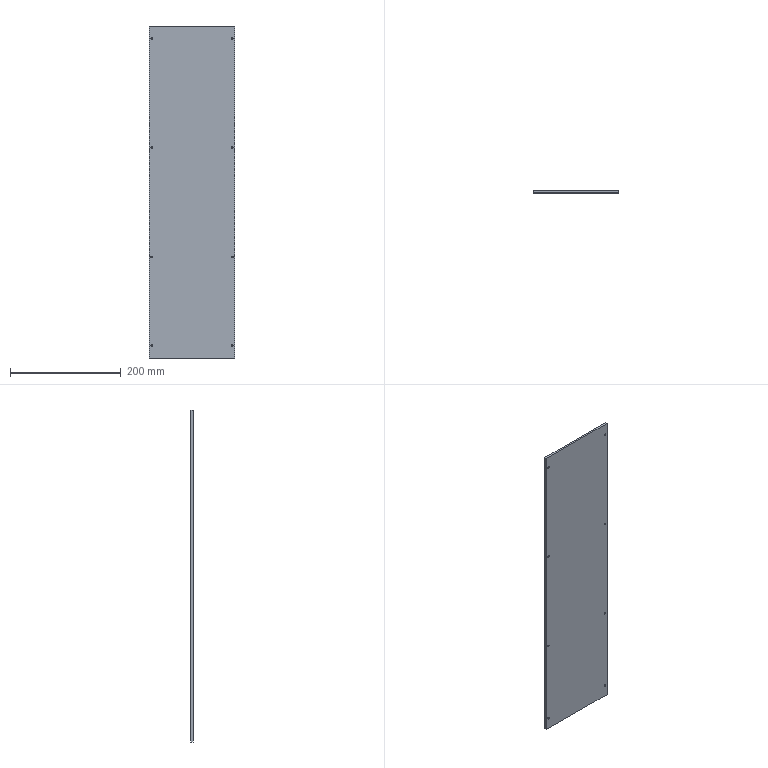Component | SolidWorks | ColumnCover-1 | 1 solid | 38 faces | box 155 x 4 x 600 mm | volume 371585 mm3 | cone 16 | cylinder 16 | plane 6 | commonest cylinder face diameters 3.4 x16
STEP:
#1=CARTESIAN_POINT('',(47.712,61.489,84.389));
#2=VERTEX_POINT('',#1);
#3=CARTESIAN_POINT('',(47.578,61.489,84.389));
#4=VERTEX_POINT('',#3);
#5=CARTESIAN_POINT('',(47.645,61.489,84.389));
#6=DIRECTION('',(-0.,1.,0.));
#7=DIRECTION('',(-1.,0.,0.));
#8=AXIS2_PLACEMENT_3D('',#5,#6,#7);
#9=CIRCLE('',#8,0.06693);
#10=EDGE_CURVE('',#2,#4,#9,.T.);
#11=ORIENTED_EDGE('',*,*,#10,.F.);
#12=CARTESIAN_POINT('',(47.771,61.548,84.389));
#13=VERTEX_POINT('',#12);
#14=CARTESIAN_POINT('',(47.771,61.548,84.389));
#15=DIRECTION('',(0.7071,0.7071,0.));
#16=VECTOR('',#15,39.37);
#17=LINE('',#14,#16);
#18=EDGE_CURVE('',#2,#13,#17,.T.);
#19=ORIENTED_EDGE('',*,*,#18,.T.);
#20=CARTESIAN_POINT('',(47.519,61.548,84.389));
#21=VERTEX_POINT('',#20);
#22=CARTESIAN_POINT('',(47.645,61.548,84.389));
#23=DIRECTION('',(-0.,1.,0.));
#24=DIRECTION('',(-1.,0.,0.));
#25=AXIS2_PLACEMENT_3D('',#22,#23,#24);
#26=CIRCLE('',#25,0.126);
#27=EDGE_CURVE('',#13,#21,#26,.T.);
#28=ORIENTED_EDGE('',*,*,#27,.T.);
#29=CARTESIAN_POINT('',(47.519,61.548,84.389));
#30=DIRECTION('',(-0.7071,0.7071,0.));
#31=VECTOR('',#30,39.37);
#32=LINE('',#29,#31);
#33=EDGE_CURVE('',#4,#21,#32,.T.);
#34=ORIENTED_EDGE('',*,*,#33,.F.);
#35=EDGE_LOOP('',(#11,#19,#28,#34));
#36=FACE_OUTER_BOUND('',#35,.T.);
#37=CARTESIAN_POINT('',(47.645,61.548,84.389));
#38=DIRECTION('',(-0.,1.,0.));
#39=DIRECTION('',(-1.,0.,0.));
#40=AXIS2_PLACEMENT_3D('',#37,#38,#39);
#41=CONICAL_SURFACE('',#40,0.126,0.7854);
#42=ADVANCED_FACE('',(#36),#41,.F.);
#43=CARTESIAN_POINT('',(47.578,61.39,84.389));
#44=VERTEX_POINT('',#43);
#45=CARTESIAN_POINT('',(47.712,61.39,84.389));
#46=VERTEX_POINT('',#45);
#47=CARTESIAN_POINT('',(47.645,61.39,84.389));
#48=DIRECTION('',(0.,-1.,-0.));
#49=DIRECTION('',(1.,0.,0.));
#50=AXIS2_PLACEMENT_3D('',#47,#48,#49);
#51=CIRCLE('',#50,0.06693);
#52=EDGE_CURVE('',#44,#46,#51,.T.);
#53=ORIENTED_EDGE('',*,*,#52,.T.);
#54=CARTESIAN_POINT('',(47.712,61.548,84.389));
#55=DIRECTION('',(-0.,1.,0.));
#56=VECTOR('',#55,39.37);
#57=LINE('',#54,#56);
#58=EDGE_CURVE('',#46,#2,#57,.T.);
#59=ORIENTED_EDGE('',*,*,#58,.T.);
#60=ORIENTED_EDGE('',*,*,#10,.T.);
#61=CARTESIAN_POINT('',(47.578,61.548,84.389));
#62=DIRECTION('',(-0.,1.,0.));
#63=VECTOR('',#62,39.37);
#64=LINE('',#61,#63);
#65=EDGE_CURVE('',#44,#4,#64,.T.);
#66=ORIENTED_EDGE('',*,*,#65,.F.);
#67=EDGE_LOOP('',(#53,#59,#60,#66));
#68=FACE_OUTER_BOUND('',#67,.T.);
#69=CARTESIAN_POINT('',(47.645,61.548,84.389));
#70=DIRECTION('',(-0.,1.,0.));
#71=DIRECTION('',(-1.,0.,0.));
#72=AXIS2_PLACEMENT_3D('',#69,#70,#71);
#73=CYLINDRICAL_SURFACE('',#72,0.06693);
#74=ADVANCED_FACE('',(#68),#73,.F.);
#75=CARTESIAN_POINT('',(42.003,61.489,84.389));
#76=VERTEX_POINT('',#75);
#77=CARTESIAN_POINT('',(41.87,61.489,84.389));
#78=VERTEX_POINT('',#77);
#79=CARTESIAN_POINT('',(41.936,61.489,84.389));
#80=DIRECTION('',(-0.,1.,0.));
#81=DIRECTION('',(-1.,0.,0.));
#82=AXIS2_PLACEMENT_3D('',#79,#80,#81);
#83=CIRCLE('',#82,0.06693);
#84=EDGE_CURVE('',#76,#78,#83,.T.);
#85=ORIENTED_EDGE('',*,*,#84,.F.);
#86=CARTESIAN_POINT('',(42.062,61.548,84.389));
#87=VERTEX_POINT('',#86);
#88=CARTESIAN_POINT('',(42.062,61.548,84.389));
#89=DIRECTION('',(0.7071,0.7071,0.));
#90=VECTOR('',#89,39.37);
#91=LINE('',#88,#90);
#92=EDGE_CURVE('',#76,#87,#91,.T.);
#93=ORIENTED_EDGE('',*,*,#92,.T.);
#94=CARTESIAN_POINT('',(41.81,61.548,84.389));
#95=VERTEX_POINT('',#94);
#96=CARTESIAN_POINT('',(41.936,61.548,84.389));
#97=DIRECTION('',(-0.,1.,0.));
#98=DIRECTION('',(-1.,0.,0.));
#99=AXIS2_PLACEMENT_3D('',#96,#97,#98);
#100=CIRCLE('',#99,0.126);
#101=EDGE_CURVE('',#87,#95,#100,.T.);
#102=ORIENTED_EDGE('',*,*,#101,.T.);
#103=CARTESIAN_POINT('',(41.81,61.548,84.389));
#104=DIRECTION('',(-0.7071,0.7071,0.));
#105=VECTOR('',#104,39.37);
#106=LINE('',#103,#105);
#107=EDGE_CURVE('',#78,#95,#106,.T.);
#108=ORIENTED_EDGE('',*,*,#107,.F.);
#109=EDGE_LOOP('',(#85,#93,#102,#108));
#110=FACE_OUTER_BOUND('',#109,.T.);
#111=CARTESIAN_POINT('',(41.936,61.548,84.389));
#112=DIRECTION('',(-0.,1.,0.));
#113=DIRECTION('',(-1.,0.,0.));
#114=AXIS2_PLACEMENT_3D('',#111,#112,#113);
#115=CONICAL_SURFACE('',#114,0.126,0.7854);
#116=ADVANCED_FACE('',(#110),#115,.F.);
#117=CARTESIAN_POINT('',(41.87,61.39,84.389));
#118=VERTEX_POINT('',#117);
#119=CARTESIAN_POINT('',(42.003,61.39,84.389));
#120=VERTEX_POINT('',#119);
#121=CARTESIAN_POINT('',(41.936,61.39,84.389));
#122=DIRECTION('',(0.,-1.,-0.));
#123=DIRECTION('',(1.,0.,0.));
#124=AXIS2_PLACEMENT_3D('',#121,#122,#123);
#125=CIRCLE('',#124,0.06693);
#126=EDGE_CURVE('',#118,#120,#125,.T.);
#127=ORIENTED_EDGE('',*,*,#126,.T.);
#128=CARTESIAN_POINT('',(42.003,61.548,84.389));
#129=DIRECTION('',(-0.,1.,0.));
#130=VECTOR('',#129,39.37);
#131=LINE('',#128,#130);
#132=EDGE_CURVE('',#120,#76,#131,.T.);
#133=ORIENTED_EDGE('',*,*,#132,.T.);
#134=ORIENTED_EDGE('',*,*,#84,.T.);
#135=CARTESIAN_POINT('',(41.87,61.548,84.389));
#136=DIRECTION('',(-0.,1.,0.));
#137=VECTOR('',#136,39.37);
#138=LINE('',#135,#137);
#139=EDGE_CURVE('',#118,#78,#138,.T.);
#140=ORIENTED_EDGE('',*,*,#139,.F.);
#141=EDGE_LOOP('',(#127,#133,#134,#140));
#142=FACE_OUTER_BOUND('',#141,.T.);
#143=CARTESIAN_POINT('',(41.936,61.548,84.389));
#144=DIRECTION('',(-0.,1.,0.));
#145=DIRECTION('',(-1.,0.,0.));
#146=AXIS2_PLACEMENT_3D('',#143,#144,#145);
#147=CYLINDRICAL_SURFACE('',#146,0.06693);
#148=ADVANCED_FACE('',(#142),#147,.F.);
#149=CARTESIAN_POINT('',(47.712,61.489,76.614));
#150=VERTEX_POINT('',#149);
#151=CARTESIAN_POINT('',(47.578,61.489,76.614));
#152=VERTEX_POINT('',#151);
#153=CARTESIAN_POINT('',(47.645,61.489,76.614));
#154=DIRECTION('',(-0.,1.,0.));
#155=DIRECTION('',(-1.,0.,0.));
#156=AXIS2_PLACEMENT_3D('',#153,#154,#155);
#157=CIRCLE('',#156,0.06693);
#158=EDGE_CURVE('',#150,#152,#157,.T.);
#159=ORIENTED_EDGE('',*,*,#158,.F.);
#160=CARTESIAN_POINT('',(47.771,61.548,76.614));
#161=VERTEX_POINT('',#160);
#162=CARTESIAN_POINT('',(47.771,61.548,76.614));
#163=DIRECTION('',(0.7071,0.7071,0.));
#164=VECTOR('',#163,39.37);
#165=LINE('',#162,#164);
#166=EDGE_CURVE('',#150,#161,#165,.T.);
#167=ORIENTED_EDGE('',*,*,#166,.T.);
#168=CARTESIAN_POINT('',(47.519,61.548,76.614));
#169=VERTEX_POINT('',#168);
#170=CARTESIAN_POINT('',(47.645,61.548,76.614));
#171=DIRECTION('',(-0.,1.,0.));
#172=DIRECTION('',(-1.,0.,0.));
#173=AXIS2_PLACEMENT_3D('',#170,#171,#172);
#174=CIRCLE('',#173,0.126);
#175=EDGE_CURVE('',#161,#169,#174,.T.);
#176=ORIENTED_EDGE('',*,*,#175,.T.);
#177=CARTESIAN_POINT('',(47.519,61.548,76.614));
#178=DIRECTION('',(-0.7071,0.7071,0.));
#179=VECTOR('',#178,39.37);
#180=LINE('',#177,#179);
#181=EDGE_CURVE('',#152,#169,#180,.T.);
#182=ORIENTED_EDGE('',*,*,#181,.F.);
#183=EDGE_LOOP('',(#159,#167,#176,#182));
#184=FACE_OUTER_BOUND('',#183,.T.);
#185=CARTESIAN_POINT('',(47.645,61.548,76.614));
#186=DIRECTION('',(-0.,1.,0.));
#187=DIRECTION('',(-1.,0.,0.));
#188=AXIS2_PLACEMENT_3D('',#185,#186,#187);
#189=CONICAL_SURFACE('',#188,0.126,0.7854);
#190=ADVANCED_FACE('',(#184),#189,.F.);
#191=CARTESIAN_POINT('',(47.578,61.39,76.614));
#192=VERTEX_POINT('',#191);
#193=CARTESIAN_POINT('',(47.712,61.39,76.614));
#194=VERTEX_POINT('',#193);
#195=CARTESIAN_POINT('',(47.645,61.39,76.614));
#196=DIRECTION('',(0.,-1.,-0.));
#197=DIRECTION('',(1.,0.,0.));
#198=AXIS2_PLACEMENT_3D('',#195,#196,#197);
#199=CIRCLE('',#198,0.06693);
#200=EDGE_CURVE('',#192,#194,#199,.T.);
#201=ORIENTED_EDGE('',*,*,#200,.T.);
#202=CARTESIAN_POINT('',(47.712,61.548,76.614));
#203=DIRECTION('',(-0.,1.,0.));
#204=VECTOR('',#203,39.37);
#205=LINE('',#202,#204);
#206=EDGE_CURVE('',#194,#150,#205,.T.);
#207=ORIENTED_EDGE('',*,*,#206,.T.);
#208=ORIENTED_EDGE('',*,*,#158,.T.);
#209=CARTESIAN_POINT('',(47.578,61.548,76.614));
#210=DIRECTION('',(-0.,1.,0.));
#211=VECTOR('',#210,39.37);
#212=LINE('',#209,#211);
#213=EDGE_CURVE('',#192,#152,#212,.T.);
#214=ORIENTED_EDGE('',*,*,#213,.F.);
#215=EDGE_LOOP('',(#201,#207,#208,#214));
#216=FACE_OUTER_BOUND('',#215,.T.);
#217=CARTESIAN_POINT('',(47.645,61.548,76.614));
#218=DIRECTION('',(-0.,1.,0.));
#219=DIRECTION('',(-1.,0.,0.));
#220=AXIS2_PLACEMENT_3D('',#217,#218,#219);
#221=CYLINDRICAL_SURFACE('',#220,0.06693);
#222=ADVANCED_FACE('',(#216),#221,.F.);
#223=CARTESIAN_POINT('',(42.003,61.489,76.614));
#224=VERTEX_POINT('',#223);
#225=CARTESIAN_POINT('',(41.87,61.489,76.614));
#226=VERTEX_POINT('',#225);
#227=CARTESIAN_POINT('',(41.936,61.489,76.614));
#228=DIRECTION('',(-0.,1.,0.));
#229=DIRECTION('',(-1.,0.,0.));
#230=AXIS2_PLACEMENT_3D('',#227,#228,#229);
#231=CIRCLE('',#230,0.06693);
#232=EDGE_CURVE('',#224,#226,#231,.T.);
#233=ORIENTED_EDGE('',*,*,#232,.F.);
#234=CARTESIAN_POINT('',(42.062,61.548,76.614));
#235=VERTEX_POINT('',#234);
#236=CARTESIAN_POINT('',(42.062,61.548,76.614));
#237=DIRECTION('',(0.7071,0.7071,0.));
#238=VECTOR('',#237,39.37);
#239=LINE('',#236,#238);
#240=EDGE_CURVE('',#224,#235,#239,.T.);
#241=ORIENTED_EDGE('',*,*,#240,.T.);
#242=CARTESIAN_POINT('',(41.81,61.548,76.614));
#243=VERTEX_POINT('',#242);
#244=CARTESIAN_POINT('',(41.936,61.548,76.614));
#245=DIRECTION('',(-0.,1.,0.));
#246=DIRECTION('',(-1.,0.,0.));
#247=AXIS2_PLACEMENT_3D('',#244,#245,#246);
#248=CIRCLE('',#247,0.126);
#249=EDGE_CURVE('',#235,#243,#248,.T.);
#250=ORIENTED_EDGE('',*,*,#249,.T.);
#251=CARTESIAN_POINT('',(41.81,61.548,76.614));
#252=DIRECTION('',(-0.7071,0.7071,0.));
#253=VECTOR('',#252,39.37);
#254=LINE('',#251,#253);
#255=EDGE_CURVE('',#226,#243,#254,.T.);
#256=ORIENTED_EDGE('',*,*,#255,.F.);
#257=EDGE_LOOP('',(#233,#241,#250,#256));
#258=FACE_OUTER_BOUND('',#257,.T.);
#259=CARTESIAN_POINT('',(41.936,61.548,76.614));
#260=DIRECTION('',(-0.,1.,0.));
#261=DIRECTION('',(-1.,0.,0.));
#262=AXIS2_PLACEMENT_3D('',#259,#260,#261);
#263=CONICAL_SURFACE('',#262,0.126,0.7854);
#264=ADVANCED_FACE('',(#258),#263,.F.);
#265=CARTESIAN_POINT('',(41.87,61.39,76.614));
#266=VERTEX_POINT('',#265);
#267=CARTESIAN_POINT('',(42.003,61.39,76.614));
#268=VERTEX_POINT('',#267);
#269=CARTESIAN_POINT('',(41.936,61.39,76.614));
#270=DIRECTION('',(0.,-1.,-0.));
#271=DIRECTION('',(1.,0.,0.));
#272=AXIS2_PLACEMENT_3D('',#269,#270,#271);
#273=CIRCLE('',#272,0.06693);
#274=EDGE_CURVE('',#266,#268,#273,.T.);
#275=ORIENTED_EDGE('',*,*,#274,.T.);
#276=CARTESIAN_POINT('',(42.003,61.548,76.614));
#277=DIRECTION('',(-0.,1.,0.));
#278=VECTOR('',#277,39.37);
#279=LINE('',#276,#278);
#280=EDGE_CURVE('',#268,#224,#279,.T.);
#281=ORIENTED_EDGE('',*,*,#280,.T.);
#282=ORIENTED_EDGE('',*,*,#232,.T.);
#283=CARTESIAN_POINT('',(41.87,61.548,76.614));
#284=DIRECTION('',(-0.,1.,0.));
#285=VECTOR('',#284,39.37);
#286=LINE('',#283,#285);
#287=EDGE_CURVE('',#266,#226,#286,.T.);
#288=ORIENTED_EDGE('',*,*,#287,.F.);
#289=EDGE_LOOP('',(#275,#281,#282,#288));
#290=FACE_OUTER_BOUND('',#289,.T.);
#291=CARTESIAN_POINT('',(41.936,61.548,76.614));
#292=DIRECTION('',(-0.,1.,0.));
#293=DIRECTION('',(-1.,0.,0.));
#294=AXIS2_PLACEMENT_3D('',#291,#292,#293);
#295=CYLINDRICAL_SURFACE('',#294,0.06693);
#296=ADVANCED_FACE('',(#290),#295,.F.);
#297=CARTESIAN_POINT('',(47.712,61.489,68.838));
#298=VERTEX_POINT('',#297);
#299=CARTESIAN_POINT('',(47.578,61.489,68.838));
#300=VERTEX_POINT('',#299);
#301=CARTESIAN_POINT('',(47.645,61.489,68.838));
#302=DIRECTION('',(-0.,1.,0.));
#303=DIRECTION('',(-1.,0.,0.));
#304=AXIS2_PLACEMENT_3D('',#301,#302,#303);
#305=CIRCLE('',#304,0.06693);
#306=EDGE_CURVE('',#298,#300,#305,.T.);
#307=ORIENTED_EDGE('',*,*,#306,.F.);
#308=CARTESIAN_POINT('',(47.771,61.548,68.838));
#309=VERTEX_POINT('',#308);
#310=CARTESIAN_POINT('',(47.771,61.548,68.838));
#311=DIRECTION('',(0.7071,0.7071,0.));
#312=VECTOR('',#311,39.37);
#313=LINE('',#310,#312);
#314=EDGE_CURVE('',#298,#309,#313,.T.);
#315=ORIENTED_EDGE('',*,*,#314,.T.);
#316=CARTESIAN_POINT('',(47.519,61.548,68.838));
#317=VERTEX_POINT('',#316);
#318=CARTESIAN_POINT('',(47.645,61.548,68.838));
#319=DIRECTION('',(-0.,1.,0.));
#320=DIRECTION('',(-1.,0.,0.));
#321=AXIS2_PLACEMENT_3D('',#318,#319,#320);
#322=CIRCLE('',#321,0.126);
#323=EDGE_CURVE('',#309,#317,#322,.T.);
#324=ORIENTED_EDGE('',*,*,#323,.T.);
#325=CARTESIAN_POINT('',(47.519,61.548,68.838));
#326=DIRECTION('',(-0.7071,0.7071,0.));
#327=VECTOR('',#326,39.37);
#328=LINE('',#325,#327);
#329=EDGE_CURVE('',#300,#317,#328,.T.);
#330=ORIENTED_EDGE('',*,*,#329,.F.);
#331=EDGE_LOOP('',(#307,#315,#324,#330));
#332=FACE_OUTER_BOUND('',#331,.T.);
#333=CARTESIAN_POINT('',(47.645,61.548,68.838));
#334=DIRECTION('',(-0.,1.,0.));
#335=DIRECTION('',(-1.,0.,0.));
#336=AXIS2_PLACEMENT_3D('',#333,#334,#335);
#337=CONICAL_SURFACE('',#336,0.126,0.7854);
#338=ADVANCED_FACE('',(#332),#337,.F.);
#339=CARTESIAN_POINT('',(47.578,61.39,68.838));
#340=VERTEX_POINT('',#339);
#341=CARTESIAN_POINT('',(47.712,61.39,68.838));
#342=VERTEX_POINT('',#341);
#343=CARTESIAN_POINT('',(47.645,61.39,68.838));
#344=DIRECTION('',(0.,-1.,-0.));
#345=DIRECTION('',(1.,0.,0.));
#346=AXIS2_PLACEMENT_3D('',#343,#344,#345);
#347=CIRCLE('',#346,0.06693);
#348=EDGE_CURVE('',#340,#342,#347,.T.);
#349=ORIENTED_EDGE('',*,*,#348,.T.);
#350=CARTESIAN_POINT('',(47.712,61.548,68.838));
#351=DIRECTION('',(-0.,1.,0.));
#352=VECTOR('',#351,39.37);
#353=LINE('',#350,#352);
#354=EDGE_CURVE('',#342,#298,#353,.T.);
#355=ORIENTED_EDGE('',*,*,#354,.T.);
#356=ORIENTED_EDGE('',*,*,#306,.T.);
#357=CARTESIAN_POINT('',(47.578,61.548,68.838));
#358=DIRECTION('',(-0.,1.,0.));
#359=VECTOR('',#358,39.37);
#360=LINE('',#357,#359);
#361=EDGE_CURVE('',#340,#300,#360,.T.);
#362=ORIENTED_EDGE('',*,*,#361,.F.);
#363=EDGE_LOOP('',(#349,#355,#356,#362));
#364=FACE_OUTER_BOUND('',#363,.T.);
#365=CARTESIAN_POINT('',(47.645,61.548,68.838));
#366=DIRECTION('',(-0.,1.,0.));
#367=DIRECTION('',(-1.,0.,0.));
#368=AXIS2_PLACEMENT_3D('',#365,#366,#367);
#369=CYLINDRICAL_SURFACE('',#368,0.06693);
#370=ADVANCED_FACE('',(#364),#369,.F.);
#371=CARTESIAN_POINT('',(42.003,61.489,68.838));
#372=VERTEX_POINT('',#371);
#373=CARTESIAN_POINT('',(41.87,61.489,68.838));
#374=VERTEX_POINT('',#373);
#375=CARTESIAN_POINT('',(41.936,61.489,68.838));
#376=DIRECTION('',(-0.,1.,0.));
#377=DIRECTION('',(-1.,0.,0.));
#378=AXIS2_PLACEMENT_3D('',#375,#376,#377);
#379=CIRCLE('',#378,0.06693);
#380=EDGE_CURVE('',#372,#374,#379,.T.);
#381=ORIENTED_EDGE('',*,*,#380,.F.);
#382=CARTESIAN_POINT('',(42.062,61.548,68.838));
#383=VERTEX_POINT('',#382);
#384=CARTESIAN_POINT('',(42.062,61.548,68.838));
#385=DIRECTION('',(0.7071,0.7071,0.));
#386=VECTOR('',#385,39.37);
#387=LINE('',#384,#386);
#388=EDGE_CURVE('',#372,#383,#387,.T.);
#389=ORIENTED_EDGE('',*,*,#388,.T.);
#390=CARTESIAN_POINT('',(41.81,61.548,68.838));
#391=VERTEX_POINT('',#390);
#392=CARTESIAN_POINT('',(41.936,61.548,68.838));
#393=DIRECTION('',(-0.,1.,0.));
#394=DIRECTION('',(-1.,0.,0.));
#395=AXIS2_PLACEMENT_3D('',#392,#393,#394);
#396=CIRCLE('',#395,0.126);
#397=EDGE_CURVE('',#383,#391,#396,.T.);
#398=ORIENTED_EDGE('',*,*,#397,.T.);
#399=CARTESIAN_POINT('',(41.81,61.548,68.838));
#400=DIRECTION('',(-0.7071,0.7071,0.));
#401=VECTOR('',#400,39.37);
#402=LINE('',#399,#401);
#403=EDGE_CURVE('',#374,#391,#402,.T.);
#404=ORIENTED_EDGE('',*,*,#403,.F.);
#405=EDGE_LOOP('',(#381,#389,#398,#404));
#406=FACE_OUTER_BOUND('',#405,.T.);
#407=CARTESIAN_POINT('',(41.936,61.548,68.838));
#408=DIRECTION('',(-0.,1.,0.));
#409=DIRECTION('',(-1.,0.,0.));
#410=AXIS2_PLACEMENT_3D('',#407,#408,#409);
#411=CONICAL_SURFACE('',#410,0.126,0.7854);
#412=ADVANCED_FACE('',(#406),#411,.F.);
#413=CARTESIAN_POINT('',(41.87,61.39,68.838));
#414=VERTEX_POINT('',#413);
#415=CARTESIAN_POINT('',(42.003,61.39,68.838));
#416=VERTEX_POINT('',#415);
#417=CARTESIAN_POINT('',(41.936,61.39,68.838));
#418=DIRECTION('',(0.,-1.,-0.));
#419=DIRECTION('',(1.,0.,0.));
#420=AXIS2_PLACEMENT_3D('',#417,#418,#419);
#421=CIRCLE('',#420,0.06693);
#422=EDGE_CURVE('',#414,#416,#421,.T.);
#423=ORIENTED_EDGE('',*,*,#422,.T.);
#424=CARTESIAN_POINT('',(42.003,61.548,68.838));
#425=DIRECTION('',(-0.,1.,0.));
#426=VECTOR('',#425,39.37);
#427=LINE('',#424,#426);
#428=EDGE_CURVE('',#416,#372,#427,.T.);
#429=ORIENTED_EDGE('',*,*,#428,.T.);
#430=ORIENTED_EDGE('',*,*,#380,.T.);
#431=CARTESIAN_POINT('',(41.87,61.548,68.838));
#432=DIRECTION('',(-0.,1.,0.));
#433=VECTOR('',#432,39.37);
#434=LINE('',#431,#433);
#435=EDGE_CURVE('',#414,#374,#434,.T.);
#436=ORIENTED_EDGE('',*,*,#435,.F.);
#437=EDGE_LOOP('',(#423,#429,#430,#436));
#438=FACE_OUTER_BOUND('',#437,.T.);
#439=CARTESIAN_POINT('',(41.936,61.548,68.838));
#440=DIRECTION('',(-0.,1.,0.));
#441=DIRECTION('',(-1.,0.,0.));
#442=AXIS2_PLACEMENT_3D('',#439,#440,#441);
#443=CYLINDRICAL_SURFACE('',#442,0.06693);
#444=ADVANCED_FACE('',(#438),#443,.F.);
#445=CARTESIAN_POINT('',(47.712,61.489,62.539));
#446=VERTEX_POINT('',#445);
#447=CARTESIAN_POINT('',(47.578,61.489,62.539));
#448=VERTEX_POINT('',#447);
#449=CARTESIAN_POINT('',(47.645,61.489,62.539));
#450=DIRECTION('',(-0.,1.,0.));
#451=DIRECTION('',(-1.,0.,0.));
#452=AXIS2_PLACEMENT_3D('',#449,#450,#451);
#453=CIRCLE('',#452,0.06693);
#454=EDGE_CURVE('',#446,#448,#453,.T.);
#455=ORIENTED_EDGE('',*,*,#454,.F.);
#456=CARTESIAN_POINT('',(47.771,61.548,62.539));
#457=VERTEX_POINT('',#456);
#458=CARTESIAN_POINT('',(47.771,61.548,62.539));
#459=DIRECTION('',(0.7071,0.7071,0.));
#460=VECTOR('',#459,39.37);
#461=LINE('',#458,#460);
#462=EDGE_CURVE('',#446,#457,#461,.T.);
#463=ORIENTED_EDGE('',*,*,#462,.T.);
#464=CARTESIAN_POINT('',(47.519,61.548,62.539));
#465=VERTEX_POINT('',#464);
#466=CARTESIAN_POINT('',(47.645,61.548,62.539));
#467=DIRECTION('',(-0.,1.,0.));
#468=DIRECTION('',(-1.,0.,0.));
#469=AXIS2_PLACEMENT_3D('',#466,#467,#468);
#470=CIRCLE('',#469,0.126);
#471=EDGE_CURVE('',#457,#465,#470,.T.);
#472=ORIENTED_EDGE('',*,*,#471,.T.);
#473=CARTESIAN_POINT('',(47.519,61.548,62.539));
#474=DIRECTION('',(-0.7071,0.7071,0.));
#475=VECTOR('',#474,39.37);
#476=LINE('',#473,#475);
#477=EDGE_CURVE('',#448,#465,#476,.T.);
#478=ORIENTED_EDGE('',*,*,#477,.F.);
#479=EDGE_LOOP('',(#455,#463,#472,#478));
#480=FACE_OUTER_BOUND('',#479,.T.);
#481=CARTESIAN_POINT('',(47.645,61.548,62.539));
#482=DIRECTION('',(-0.,1.,0.));
#483=DIRECTION('',(-1.,0.,0.));
#484=AXIS2_PLACEMENT_3D('',#481,#482,#483);
#485=CONICAL_SURFACE('',#484,0.126,0.7854);
#486=ADVANCED_FACE('',(#480),#485,.F.);
#487=CARTESIAN_POINT('',(47.578,61.39,62.539));
#488=VERTEX_POINT('',#487);
#489=CARTESIAN_POINT('',(47.712,61.39,62.539));
#490=VERTEX_POINT('',#489);
#491=CARTESIAN_POINT('',(47.645,61.39,62.539));
#492=DIRECTION('',(0.,-1.,-0.));
#493=DIRECTION('',(1.,0.,0.));
#494=AXIS2_PLACEMENT_3D('',#491,#492,#493);
#495=CIRCLE('',#494,0.06693);
#496=EDGE_CURVE('',#488,#490,#495,.T.);
#497=ORIENTED_EDGE('',*,*,#496,.T.);
#498=CARTESIAN_POINT('',(47.712,61.548,62.539));
#499=DIRECTION('',(-0.,1.,0.));
#500=VECTOR('',#499,39.37);
#501=LINE('',#498,#500);
#502=EDGE_CURVE('',#490,#446,#501,.T.);
#503=ORIENTED_EDGE('',*,*,#502,.T.);
#504=ORIENTED_EDGE('',*,*,#454,.T.);
#505=CARTESIAN_POINT('',(47.578,61.548,62.539));
#506=DIRECTION('',(-0.,1.,0.));
#507=VECTOR('',#506,39.37);
#508=LINE('',#505,#507);
#509=EDGE_CURVE('',#488,#448,#508,.T.);
#510=ORIENTED_EDGE('',*,*,#509,.F.);
#511=EDGE_LOOP('',(#497,#503,#504,#510));
#512=FACE_OUTER_BOUND('',#511,.T.);
#513=CARTESIAN_POINT('',(47.645,61.548,62.539));
#514=DIRECTION('',(-0.,1.,0.));
#515=DIRECTION('',(-1.,0.,0.));
#516=AXIS2_PLACEMENT_3D('',#513,#514,#515);
#517=CYLINDRICAL_SURFACE('',#516,0.06693);
#518=ADVANCED_FACE('',(#512),#517,.F.);
#519=CARTESIAN_POINT('',(42.003,61.489,62.539));
#520=VERTEX_POINT('',#519);
#521=CARTESIAN_POINT('',(41.87,61.489,62.539));
#522=VERTEX_POINT('',#521);
#523=CARTESIAN_POINT('',(41.936,61.489,62.539));
#524=DIRECTION('',(-0.,1.,0.));
#525=DIRECTION('',(-1.,0.,0.));
#526=AXIS2_PLACEMENT_3D('',#523,#524,#525);
#527=CIRCLE('',#526,0.06693);
#528=EDGE_CURVE('',#520,#522,#527,.T.);
#529=ORIENTED_EDGE('',*,*,#528,.F.);
#530=CARTESIAN_POINT('',(42.062,61.548,62.539));
#531=VERTEX_POINT('',#530);
#532=CARTESIAN_POINT('',(42.062,61.548,62.539));
#533=DIRECTION('',(0.7071,0.7071,0.));
#534=VECTOR('',#533,39.37);
#535=LINE('',#532,#534);
#536=EDGE_CURVE('',#520,#531,#535,.T.);
#537=ORIENTED_EDGE('',*,*,#536,.T.);
#538=CARTESIAN_POINT('',(41.81,61.548,62.539));
#539=VERTEX_POINT('',#538);
#540=CARTESIAN_POINT('',(41.936,61.548,62.539));
#541=DIRECTION('',(-0.,1.,0.));
#542=DIRECTION('',(-1.,0.,0.));
#543=AXIS2_PLACEMENT_3D('',#540,#541,#542);
#544=CIRCLE('',#543,0.126);
#545=EDGE_CURVE('',#531,#539,#544,.T.);
#546=ORIENTED_EDGE('',*,*,#545,.T.);
#547=CARTESIAN_POINT('',(41.81,61.548,62.539));
#548=DIRECTION('',(-0.7071,0.7071,0.));
#549=VECTOR('',#548,39.37);
#550=LINE('',#547,#549);
#551=EDGE_CURVE('',#522,#539,#550,.T.);
#552=ORIENTED_EDGE('',*,*,#551,.F.);
#553=EDGE_LOOP('',(#529,#537,#546,#552));
#554=FACE_OUTER_BOUND('',#553,.T.);
#555=CARTESIAN_POINT('',(41.936,61.548,62.539));
#556=DIRECTION('',(-0.,1.,0.));
#557=DIRECTION('',(-1.,0.,0.));
#558=AXIS2_PLACEMENT_3D('',#555,#556,#557);
#559=CONICAL_SURFACE('',#558,0.126,0.7854);
#560=ADVANCED_FACE('',(#554),#559,.F.);
#561=CARTESIAN_POINT('',(41.87,61.39,62.539));
#562=VERTEX_POINT('',#561);
#563=CARTESIAN_POINT('',(42.003,61.39,62.539));
#564=VERTEX_POINT('',#563);
#565=CARTESIAN_POINT('',(41.936,61.39,62.539));
#566=DIRECTION('',(0.,-1.,-0.));
#567=DIRECTION('',(1.,0.,0.));
#568=AXIS2_PLACEMENT_3D('',#565,#566,#567);
#569=CIRCLE('',#568,0.06693);
#570=EDGE_CURVE('',#562,#564,#569,.T.);
#571=ORIENTED_EDGE('',*,*,#570,.T.);
#572=CARTESIAN_POINT('',(42.003,61.548,62.539));
#573=DIRECTION('',(-0.,1.,0.));
#574=VECTOR('',#573,39.37);
#575=LINE('',#572,#574);
#576=EDGE_CURVE('',#564,#520,#575,.T.);
#577=ORIENTED_EDGE('',*,*,#576,.T.);
#578=ORIENTED_EDGE('',*,*,#528,.T.);
#579=CARTESIAN_POINT('',(41.87,61.548,62.539));
#580=DIRECTION('',(-0.,1.,0.));
#581=VECTOR('',#580,39.37);
#582=LINE('',#579,#581);
#583=EDGE_CURVE('',#562,#522,#582,.T.);
#584=ORIENTED_EDGE('',*,*,#583,.F.);
#585=EDGE_LOOP('',(#571,#577,#578,#584));
#586=FACE_OUTER_BOUND('',#585,.T.);
#587=CARTESIAN_POINT('',(41.936,61.548,62.539));
#588=DIRECTION('',(-0.,1.,0.));
#589=DIRECTION('',(-1.,0.,0.));
#590=AXIS2_PLACEMENT_3D('',#587,#588,#589);
#591=CYLINDRICAL_SURFACE('',#590,0.06693);
#592=ADVANCED_FACE('',(#586),#591,.F.);
#593=CARTESIAN_POINT('',(41.74,61.39,61.653));
#594=VERTEX_POINT('',#593);
#595=CARTESIAN_POINT('',(41.74,61.39,85.275));
#596=VERTEX_POINT('',#595);
#597=CARTESIAN_POINT('',(41.74,61.39,61.653));
#598=DIRECTION('',(0.,-0.,1.));
#599=VECTOR('',#598,39.37);
#600=LINE('',#597,#599);
#601=EDGE_CURVE('',#594,#596,#600,.T.);
#602=ORIENTED_EDGE('',*,*,#601,.T.);
#603=CARTESIAN_POINT('',(41.74,61.548,85.275));
#604=VERTEX_POINT('',#603);
#605=CARTESIAN_POINT('',(41.74,61.548,85.275));
#606=DIRECTION('',(0.,-1.,-0.));
#607=VECTOR('',#606,39.37);
#608=LINE('',#605,#607);
#609=EDGE_CURVE('',#604,#596,#608,.T.);
#610=ORIENTED_EDGE('',*,*,#609,.F.);
#611=CARTESIAN_POINT('',(41.74,61.548,61.653));
#612=VERTEX_POINT('',#611);
#613=CARTESIAN_POINT('',(41.74,61.548,61.653));
#614=DIRECTION('',(0.,-0.,1.));
#615=VECTOR('',#614,39.37);
#616=LINE('',#613,#615);
#617=EDGE_CURVE('',#612,#604,#616,.T.);
#618=ORIENTED_EDGE('',*,*,#617,.F.);
#619=CARTESIAN_POINT('',(41.74,61.548,61.653));
#620=DIRECTION('',(0.,-1.,-0.));
#621=VECTOR('',#620,39.37);
#622=LINE('',#619,#621);
#623=EDGE_CURVE('',#612,#594,#622,.T.);
#624=ORIENTED_EDGE('',*,*,#623,.T.);
#625=EDGE_LOOP('',(#602,#610,#618,#624));
#626=FACE_OUTER_BOUND('',#625,.T.);
#627=CARTESIAN_POINT('',(41.74,61.548,61.653));
#628=DIRECTION('',(1.,0.,0.));
#629=DIRECTION('',(-0.,1.,0.));
#630=AXIS2_PLACEMENT_3D('',#627,#628,#629);
#631=PLANE('',#630);
#632=ADVANCED_FACE('',(#626),#631,.F.);
#633=CARTESIAN_POINT('',(47.842,61.39,85.275));
#634=VERTEX_POINT('',#633);
#635=CARTESIAN_POINT('',(47.842,61.39,85.275));
#636=DIRECTION('',(1.,-0.,0.));
#637=VECTOR('',#636,39.37);
#638=LINE('',#635,#637);
#639=EDGE_CURVE('',#596,#634,#638,.T.);
#640=ORIENTED_EDGE('',*,*,#639,.T.);
#641=CARTESIAN_POINT('',(47.842,61.548,85.275));
#642=VERTEX_POINT('',#641);
#643=CARTESIAN_POINT('',(47.842,61.548,85.275));
#644=DIRECTION('',(0.,-1.,-0.));
#645=VECTOR('',#644,39.37);
#646=LINE('',#643,#645);
#647=EDGE_CURVE('',#642,#634,#646,.T.);
#648=ORIENTED_EDGE('',*,*,#647,.F.);
#649=CARTESIAN_POINT('',(47.842,61.548,85.275));
#650=DIRECTION('',(1.,-0.,0.));
#651=VECTOR('',#650,39.37);
#652=LINE('',#649,#651);
#653=EDGE_CURVE('',#604,#642,#652,.T.);
#654=ORIENTED_EDGE('',*,*,#653,.F.);
#655=ORIENTED_EDGE('',*,*,#609,.T.);
#656=EDGE_LOOP('',(#640,#648,#654,#655));
#657=FACE_OUTER_BOUND('',#656,.T.);
#658=CARTESIAN_POINT('',(47.842,61.548,85.275));
#659=DIRECTION('',(-0.,0.,-1.));
#660=DIRECTION('',(0.,-1.,-0.));
#661=AXIS2_PLACEMENT_3D('',#658,#659,#660);
#662=PLANE('',#661);
#663=ADVANCED_FACE('',(#657),#662,.F.);
#664=CARTESIAN_POINT('',(47.842,61.39,61.653));
#665=VERTEX_POINT('',#664);
#666=CARTESIAN_POINT('',(47.842,61.39,61.653));
#667=DIRECTION('',(-0.,0.,-1.));
#668=VECTOR('',#667,39.37);
#669=LINE('',#666,#668);
#670=EDGE_CURVE('',#634,#665,#669,.T.);
#671=ORIENTED_EDGE('',*,*,#670,.T.);
#672=CARTESIAN_POINT('',(47.842,61.548,61.653));
#673=VERTEX_POINT('',#672);
#674=CARTESIAN_POINT('',(47.842,61.548,61.653));
#675=DIRECTION('',(0.,-1.,-0.));
#676=VECTOR('',#675,39.37);
#677=LINE('',#674,#676);
#678=EDGE_CURVE('',#673,#665,#677,.T.);
#679=ORIENTED_EDGE('',*,*,#678,.F.);
#680=CARTESIAN_POINT('',(47.842,61.548,61.653));
#681=DIRECTION('',(-0.,0.,-1.));
#682=VECTOR('',#681,39.37);
#683=LINE('',#680,#682);
#684=EDGE_CURVE('',#642,#673,#683,.T.);
#685=ORIENTED_EDGE('',*,*,#684,.F.);
#686=ORIENTED_EDGE('',*,*,#647,.T.);
#687=EDGE_LOOP('',(#671,#679,#685,#686));
#688=FACE_OUTER_BOUND('',#687,.T.);
#689=CARTESIAN_POINT('',(47.842,61.548,61.653));
#690=DIRECTION('',(-1.,-0.,-0.));
#691=DIRECTION('',(0.,-1.,-0.));
#692=AXIS2_PLACEMENT_3D('',#689,#690,#691);
#693=PLANE('',#692);
#694=ADVANCED_FACE('',(#688),#693,.F.);
#695=CARTESIAN_POINT('',(47.842,61.39,61.653));
#696=DIRECTION('',(-1.,0.,-0.));
#697=VECTOR('',#696,39.37);
#698=LINE('',#695,#697);
#699=EDGE_CURVE('',#665,#594,#698,.T.);
#700=ORIENTED_EDGE('',*,*,#699,.T.);
#701=ORIENTED_EDGE('',*,*,#623,.F.);
#702=CARTESIAN_POINT('',(47.842,61.548,61.653));
#703=DIRECTION('',(-1.,0.,-0.));
#704=VECTOR('',#703,39.37);
#705=LINE('',#702,#704);
#706=EDGE_CURVE('',#673,#612,#705,.T.);
#707=ORIENTED_EDGE('',*,*,#706,.F.);
#708=ORIENTED_EDGE('',*,*,#678,.T.);
#709=EDGE_LOOP('',(#700,#701,#707,#708));
#710=FACE_OUTER_BOUND('',#709,.T.);
#711=CARTESIAN_POINT('',(47.842,61.548,61.653));
#712=DIRECTION('',(0.,-0.,1.));
#713=DIRECTION('',(-0.,1.,0.));
#714=AXIS2_PLACEMENT_3D('',#711,#712,#713);
#715=PLANE('',#714);
#716=ADVANCED_FACE('',(#710),#715,.F.);
#717=CARTESIAN_POINT('',(47.645,61.548,84.389));
#718=DIRECTION('',(-0.,1.,0.));
#719=DIRECTION('',(-1.,0.,0.));
#720=AXIS2_PLACEMENT_3D('',#717,#718,#719);
#721=CIRCLE('',#720,0.126);
#722=EDGE_CURVE('',#21,#13,#721,.T.);
#723=ORIENTED_EDGE('',*,*,#722,.F.);
#724=ORIENTED_EDGE('',*,*,#27,.F.);
#725=EDGE_LOOP('',(#723,#724));
#726=FACE_BOUND('',#725,.T.);
#727=CARTESIAN_POINT('',(41.936,61.548,84.389));
#728=DIRECTION('',(-0.,1.,0.));
#729=DIRECTION('',(-1.,0.,0.));
#730=AXIS2_PLACEMENT_3D('',#727,#728,#729);
#731=CIRCLE('',#730,0.126);
#732=EDGE_CURVE('',#95,#87,#731,.T.);
#733=ORIENTED_EDGE('',*,*,#732,.F.);
#734=ORIENTED_EDGE('',*,*,#101,.F.);
#735=EDGE_LOOP('',(#733,#734));
#736=FACE_BOUND('',#735,.T.);
#737=CARTESIAN_POINT('',(47.645,61.548,76.614));
#738=DIRECTION('',(-0.,1.,0.));
#739=DIRECTION('',(-1.,0.,0.));
#740=AXIS2_PLACEMENT_3D('',#737,#738,#739);
#741=CIRCLE('',#740,0.126);
#742=EDGE_CURVE('',#169,#161,#741,.T.);
#743=ORIENTED_EDGE('',*,*,#742,.F.);
#744=ORIENTED_EDGE('',*,*,#175,.F.);
#745=EDGE_LOOP('',(#743,#744));
#746=FACE_BOUND('',#745,.T.);
#747=CARTESIAN_POINT('',(41.936,61.548,76.614));
#748=DIRECTION('',(-0.,1.,0.));
#749=DIRECTION('',(-1.,0.,0.));
#750=AXIS2_PLACEMENT_3D('',#747,#748,#749);
#751=CIRCLE('',#750,0.126);
#752=EDGE_CURVE('',#243,#235,#751,.T.);
#753=ORIENTED_EDGE('',*,*,#752,.F.);
#754=ORIENTED_EDGE('',*,*,#249,.F.);
#755=EDGE_LOOP('',(#753,#754));
#756=FACE_BOUND('',#755,.T.);
#757=CARTESIAN_POINT('',(47.645,61.548,68.838));
#758=DIRECTION('',(-0.,1.,0.));
#759=DIRECTION('',(-1.,0.,0.));
#760=AXIS2_PLACEMENT_3D('',#757,#758,#759);
#761=CIRCLE('',#760,0.126);
#762=EDGE_CURVE('',#317,#309,#761,.T.);
#763=ORIENTED_EDGE('',*,*,#762,.F.);
#764=ORIENTED_EDGE('',*,*,#323,.F.);
#765=EDGE_LOOP('',(#763,#764));
#766=FACE_BOUND('',#765,.T.);
#767=CARTESIAN_POINT('',(41.936,61.548,68.838));
#768=DIRECTION('',(-0.,1.,0.));
#769=DIRECTION('',(-1.,0.,0.));
#770=AXIS2_PLACEMENT_3D('',#767,#768,#769);
#771=CIRCLE('',#770,0.126);
#772=EDGE_CURVE('',#391,#383,#771,.T.);
#773=ORIENTED_EDGE('',*,*,#772,.F.);
#774=ORIENTED_EDGE('',*,*,#397,.F.);
#775=EDGE_LOOP('',(#773,#774));
#776=FACE_BOUND('',#775,.T.);
#777=CARTESIAN_POINT('',(47.645,61.548,62.539));
#778=DIRECTION('',(-0.,1.,0.));
#779=DIRECTION('',(-1.,0.,0.));
#780=AXIS2_PLACEMENT_3D('',#777,#778,#779);
#781=CIRCLE('',#780,0.126);
#782=EDGE_CURVE('',#465,#457,#781,.T.);
#783=ORIENTED_EDGE('',*,*,#782,.F.);
#784=ORIENTED_EDGE('',*,*,#471,.F.);
#785=EDGE_LOOP('',(#783,#784));
#786=FACE_BOUND('',#785,.T.);
#787=CARTESIAN_POINT('',(41.936,61.548,62.539));
#788=DIRECTION('',(-0.,1.,0.));
#789=DIRECTION('',(-1.,0.,0.));
#790=AXIS2_PLACEMENT_3D('',#787,#788,#789);
#791=CIRCLE('',#790,0.126);
#792=EDGE_CURVE('',#539,#531,#791,.T.);
#793=ORIENTED_EDGE('',*,*,#792,.F.);
#794=ORIENTED_EDGE('',*,*,#545,.F.);
#795=EDGE_LOOP('',(#793,#794));
#796=FACE_BOUND('',#795,.T.);
#797=ORIENTED_EDGE('',*,*,#617,.T.);
#798=ORIENTED_EDGE('',*,*,#653,.T.);
#799=ORIENTED_EDGE('',*,*,#684,.T.);
#800=ORIENTED_EDGE('',*,*,#706,.T.);
#801=EDGE_LOOP('',(#797,#798,#799,#800));
#802=FACE_OUTER_BOUND('',#801,.T.);
#803=CARTESIAN_POINT('',(44.791,61.548,73.464));
#804=DIRECTION('',(-0.,-1.,-0.));
#805=DIRECTION('',(1.,-0.,0.));
#806=AXIS2_PLACEMENT_3D('',#803,#804,#805);
#807=PLANE('',#806);
#808=ADVANCED_FACE('',(#726,#736,#746,#756,#766,#776,#786,#796,#802),#807,.F.);
#809=ORIENTED_EDGE('',*,*,#52,.F.);
#810=CARTESIAN_POINT('',(47.645,61.39,84.389));
#811=DIRECTION('',(0.,-1.,-0.));
#812=DIRECTION('',(1.,0.,0.));
#813=AXIS2_PLACEMENT_3D('',#810,#811,#812);
#814=CIRCLE('',#813,0.06693);
#815=EDGE_CURVE('',#46,#44,#814,.T.);
#816=ORIENTED_EDGE('',*,*,#815,.F.);
#817=EDGE_LOOP('',(#809,#816));
#818=FACE_BOUND('',#817,.T.);
#819=ORIENTED_EDGE('',*,*,#126,.F.);
#820=CARTESIAN_POINT('',(41.936,61.39,84.389));
#821=DIRECTION('',(0.,-1.,-0.));
#822=DIRECTION('',(1.,0.,0.));
#823=AXIS2_PLACEMENT_3D('',#820,#821,#822);
#824=CIRCLE('',#823,0.06693);
#825=EDGE_CURVE('',#120,#118,#824,.T.);
#826=ORIENTED_EDGE('',*,*,#825,.F.);
#827=EDGE_LOOP('',(#819,#826));
#828=FACE_BOUND('',#827,.T.);
#829=ORIENTED_EDGE('',*,*,#200,.F.);
#830=CARTESIAN_POINT('',(47.645,61.39,76.614));
#831=DIRECTION('',(0.,-1.,-0.));
#832=DIRECTION('',(1.,0.,0.));
#833=AXIS2_PLACEMENT_3D('',#830,#831,#832);
#834=CIRCLE('',#833,0.06693);
#835=EDGE_CURVE('',#194,#192,#834,.T.);
#836=ORIENTED_EDGE('',*,*,#835,.F.);
#837=EDGE_LOOP('',(#829,#836));
#838=FACE_BOUND('',#837,.T.);
#839=ORIENTED_EDGE('',*,*,#274,.F.);
#840=CARTESIAN_POINT('',(41.936,61.39,76.614));
#841=DIRECTION('',(0.,-1.,-0.));
#842=DIRECTION('',(1.,0.,0.));
#843=AXIS2_PLACEMENT_3D('',#840,#841,#842);
#844=CIRCLE('',#843,0.06693);
#845=EDGE_CURVE('',#268,#266,#844,.T.);
#846=ORIENTED_EDGE('',*,*,#845,.F.);
#847=EDGE_LOOP('',(#839,#846));
#848=FACE_BOUND('',#847,.T.);
#849=ORIENTED_EDGE('',*,*,#348,.F.);
#850=CARTESIAN_POINT('',(47.645,61.39,68.838));
#851=DIRECTION('',(0.,-1.,-0.));
#852=DIRECTION('',(1.,0.,0.));
#853=AXIS2_PLACEMENT_3D('',#850,#851,#852);
#854=CIRCLE('',#853,0.06693);
#855=EDGE_CURVE('',#342,#340,#854,.T.);
#856=ORIENTED_EDGE('',*,*,#855,.F.);
#857=EDGE_LOOP('',(#849,#856));
#858=FACE_BOUND('',#857,.T.);
#859=ORIENTED_EDGE('',*,*,#422,.F.);
#860=CARTESIAN_POINT('',(41.936,61.39,68.838));
#861=DIRECTION('',(0.,-1.,-0.));
#862=DIRECTION('',(1.,0.,0.));
#863=AXIS2_PLACEMENT_3D('',#860,#861,#862);
#864=CIRCLE('',#863,0.06693);
#865=EDGE_CURVE('',#416,#414,#864,.T.);
#866=ORIENTED_EDGE('',*,*,#865,.F.);
#867=EDGE_LOOP('',(#859,#866));
#868=FACE_BOUND('',#867,.T.);
#869=ORIENTED_EDGE('',*,*,#496,.F.);
#870=CARTESIAN_POINT('',(47.645,61.39,62.539));
#871=DIRECTION('',(0.,-1.,-0.));
#872=DIRECTION('',(1.,0.,0.));
#873=AXIS2_PLACEMENT_3D('',#870,#871,#872);
#874=CIRCLE('',#873,0.06693);
#875=EDGE_CURVE('',#490,#488,#874,.T.);
#876=ORIENTED_EDGE('',*,*,#875,.F.);
#877=EDGE_LOOP('',(#869,#876));
#878=FACE_BOUND('',#877,.T.);
#879=ORIENTED_EDGE('',*,*,#570,.F.);
#880=CARTESIAN_POINT('',(41.936,61.39,62.539));
#881=DIRECTION('',(0.,-1.,-0.));
#882=DIRECTION('',(1.,0.,0.));
#883=AXIS2_PLACEMENT_3D('',#880,#881,#882);
#884=CIRCLE('',#883,0.06693);
#885=EDGE_CURVE('',#564,#562,#884,.T.);
#886=ORIENTED_EDGE('',*,*,#885,.F.);
#887=EDGE_LOOP('',(#879,#886));
#888=FACE_BOUND('',#887,.T.);
#889=ORIENTED_EDGE('',*,*,#601,.F.);
#890=ORIENTED_EDGE('',*,*,#699,.F.);
#891=ORIENTED_EDGE('',*,*,#670,.F.);
#892=ORIENTED_EDGE('',*,*,#639,.F.);
#893=EDGE_LOOP('',(#889,#890,#891,#892));
#894=FACE_OUTER_BOUND('',#893,.T.);
#895=CARTESIAN_POINT('',(44.791,61.39,73.464));
#896=DIRECTION('',(-0.,-1.,-0.));
#897=DIRECTION('',(1.,-0.,0.));
#898=AXIS2_PLACEMENT_3D('',#895,#896,#897);
#899=PLANE('',#898);
#900=ADVANCED_FACE('',(#818,#828,#838,#848,#858,#868,#878,#888,#894),#899,.T.);
#901=ORIENTED_EDGE('',*,*,#576,.F.);
#902=ORIENTED_EDGE('',*,*,#885,.T.);
#903=ORIENTED_EDGE('',*,*,#583,.T.);
#904=CARTESIAN_POINT('',(41.936,61.489,62.539));
#905=DIRECTION('',(-0.,1.,0.));
#906=DIRECTION('',(-1.,0.,0.));
#907=AXIS2_PLACEMENT_3D('',#904,#905,#906);
#908=CIRCLE('',#907,0.06693);
#909=EDGE_CURVE('',#522,#520,#908,.T.);
#910=ORIENTED_EDGE('',*,*,#909,.T.);
#911=EDGE_LOOP('',(#901,#902,#903,#910));
#912=FACE_OUTER_BOUND('',#911,.T.);
#913=CARTESIAN_POINT('',(41.936,61.548,62.539));
#914=DIRECTION('',(-0.,1.,0.));
#915=DIRECTION('',(-1.,0.,0.));
#916=AXIS2_PLACEMENT_3D('',#913,#914,#915);
#917=CYLINDRICAL_SURFACE('',#916,0.06693);
#918=ADVANCED_FACE('',(#912),#917,.F.);
#919=ORIENTED_EDGE('',*,*,#536,.F.);
#920=ORIENTED_EDGE('',*,*,#909,.F.);
#921=ORIENTED_EDGE('',*,*,#551,.T.);
#922=ORIENTED_EDGE('',*,*,#792,.T.);
#923=EDGE_LOOP('',(#919,#920,#921,#922));
#924=FACE_OUTER_BOUND('',#923,.T.);
#925=CARTESIAN_POINT('',(41.936,61.548,62.539));
#926=DIRECTION('',(-0.,1.,0.));
#927=DIRECTION('',(-1.,0.,0.));
#928=AXIS2_PLACEMENT_3D('',#925,#926,#927);
#929=CONICAL_SURFACE('',#928,0.126,0.7854);
#930=ADVANCED_FACE('',(#924),#929,.F.);
#931=ORIENTED_EDGE('',*,*,#502,.F.);
#932=ORIENTED_EDGE('',*,*,#875,.T.);
#933=ORIENTED_EDGE('',*,*,#509,.T.);
#934=CARTESIAN_POINT('',(47.645,61.489,62.539));
#935=DIRECTION('',(-0.,1.,0.));
#936=DIRECTION('',(-1.,0.,0.));
#937=AXIS2_PLACEMENT_3D('',#934,#935,#936);
#938=CIRCLE('',#937,0.06693);
#939=EDGE_CURVE('',#448,#446,#938,.T.);
#940=ORIENTED_EDGE('',*,*,#939,.T.);
#941=EDGE_LOOP('',(#931,#932,#933,#940));
#942=FACE_OUTER_BOUND('',#941,.T.);
#943=CARTESIAN_POINT('',(47.645,61.548,62.539));
#944=DIRECTION('',(-0.,1.,0.));
#945=DIRECTION('',(-1.,0.,0.));
#946=AXIS2_PLACEMENT_3D('',#943,#944,#945);
#947=CYLINDRICAL_SURFACE('',#946,0.06693);
#948=ADVANCED_FACE('',(#942),#947,.F.);
#949=ORIENTED_EDGE('',*,*,#462,.F.);
#950=ORIENTED_EDGE('',*,*,#939,.F.);
#951=ORIENTED_EDGE('',*,*,#477,.T.);
#952=ORIENTED_EDGE('',*,*,#782,.T.);
#953=EDGE_LOOP('',(#949,#950,#951,#952));
#954=FACE_OUTER_BOUND('',#953,.T.);
#955=CARTESIAN_POINT('',(47.645,61.548,62.539));
#956=DIRECTION('',(-0.,1.,0.));
#957=DIRECTION('',(-1.,0.,0.));
#958=AXIS2_PLACEMENT_3D('',#955,#956,#957);
#959=CONICAL_SURFACE('',#958,0.126,0.7854);
#960=ADVANCED_FACE('',(#954),#959,.F.);
#961=ORIENTED_EDGE('',*,*,#428,.F.);
#962=ORIENTED_EDGE('',*,*,#865,.T.);
#963=ORIENTED_EDGE('',*,*,#435,.T.);
#964=CARTESIAN_POINT('',(41.936,61.489,68.838));
#965=DIRECTION('',(-0.,1.,0.));
#966=DIRECTION('',(-1.,0.,0.));
#967=AXIS2_PLACEMENT_3D('',#964,#965,#966);
#968=CIRCLE('',#967,0.06693);
#969=EDGE_CURVE('',#374,#372,#968,.T.);
#970=ORIENTED_EDGE('',*,*,#969,.T.);
#971=EDGE_LOOP('',(#961,#962,#963,#970));
#972=FACE_OUTER_BOUND('',#971,.T.);
#973=CARTESIAN_POINT('',(41.936,61.548,68.838));
#974=DIRECTION('',(-0.,1.,0.));
#975=DIRECTION('',(-1.,0.,0.));
#976=AXIS2_PLACEMENT_3D('',#973,#974,#975);
#977=CYLINDRICAL_SURFACE('',#976,0.06693);
#978=ADVANCED_FACE('',(#972),#977,.F.);
#979=ORIENTED_EDGE('',*,*,#388,.F.);
#980=ORIENTED_EDGE('',*,*,#969,.F.);
#981=ORIENTED_EDGE('',*,*,#403,.T.);
#982=ORIENTED_EDGE('',*,*,#772,.T.);
#983=EDGE_LOOP('',(#979,#980,#981,#982));
#984=FACE_OUTER_BOUND('',#983,.T.);
#985=CARTESIAN_POINT('',(41.936,61.548,68.838));
#986=DIRECTION('',(-0.,1.,0.));
#987=DIRECTION('',(-1.,0.,0.));
#988=AXIS2_PLACEMENT_3D('',#985,#986,#987);
#989=CONICAL_SURFACE('',#988,0.126,0.7854);
#990=ADVANCED_FACE('',(#984),#989,.F.);
#991=ORIENTED_EDGE('',*,*,#354,.F.);
#992=ORIENTED_EDGE('',*,*,#855,.T.);
#993=ORIENTED_EDGE('',*,*,#361,.T.);
#994=CARTESIAN_POINT('',(47.645,61.489,68.838));
#995=DIRECTION('',(-0.,1.,0.));
#996=DIRECTION('',(-1.,0.,0.));
#997=AXIS2_PLACEMENT_3D('',#994,#995,#996);
#998=CIRCLE('',#997,0.06693);
#999=EDGE_CURVE('',#300,#298,#998,.T.);
#1000=ORIENTED_EDGE('',*,*,#999,.T.);
#1001=EDGE_LOOP('',(#991,#992,#993,#1000));
#1002=FACE_OUTER_BOUND('',#1001,.T.);
#1003=CARTESIAN_POINT('',(47.645,61.548,68.838));
#1004=DIRECTION('',(-0.,1.,0.));
#1005=DIRECTION('',(-1.,0.,0.));
#1006=AXIS2_PLACEMENT_3D('',#1003,#1004,#1005);
#1007=CYLINDRICAL_SURFACE('',#1006,0.06693);
#1008=ADVANCED_FACE('',(#1002),#1007,.F.);
#1009=ORIENTED_EDGE('',*,*,#314,.F.);
#1010=ORIENTED_EDGE('',*,*,#999,.F.);
#1011=ORIENTED_EDGE('',*,*,#329,.T.);
#1012=ORIENTED_EDGE('',*,*,#762,.T.);
#1013=EDGE_LOOP('',(#1009,#1010,#1011,#1012));
#1014=FACE_OUTER_BOUND('',#1013,.T.);
#1015=CARTESIAN_POINT('',(47.645,61.548,68.838));
#1016=DIRECTION('',(-0.,1.,0.));
#1017=DIRECTION('',(-1.,0.,0.));
#1018=AXIS2_PLACEMENT_3D('',#1015,#1016,#1017);
#1019=CONICAL_SURFACE('',#1018,0.126,0.7854);
#1020=ADVANCED_FACE('',(#1014),#1019,.F.);
#1021=ORIENTED_EDGE('',*,*,#280,.F.);
#1022=ORIENTED_EDGE('',*,*,#845,.T.);
#1023=ORIENTED_EDGE('',*,*,#287,.T.);
#1024=CARTESIAN_POINT('',(41.936,61.489,76.614));
#1025=DIRECTION('',(-0.,1.,0.));
#1026=DIRECTION('',(-1.,0.,0.));
#1027=AXIS2_PLACEMENT_3D('',#1024,#1025,#1026);
#1028=CIRCLE('',#1027,0.06693);
#1029=EDGE_CURVE('',#226,#224,#1028,.T.);
#1030=ORIENTED_EDGE('',*,*,#1029,.T.);
#1031=EDGE_LOOP('',(#1021,#1022,#1023,#1030));
#1032=FACE_OUTER_BOUND('',#1031,.T.);
#1033=CARTESIAN_POINT('',(41.936,61.548,76.614));
#1034=DIRECTION('',(-0.,1.,0.));
#1035=DIRECTION('',(-1.,0.,0.));
#1036=AXIS2_PLACEMENT_3D('',#1033,#1034,#1035);
#1037=CYLINDRICAL_SURFACE('',#1036,0.06693);
#1038=ADVANCED_FACE('',(#1032),#1037,.F.);
#1039=ORIENTED_EDGE('',*,*,#240,.F.);
#1040=ORIENTED_EDGE('',*,*,#1029,.F.);
#1041=ORIENTED_EDGE('',*,*,#255,.T.);
#1042=ORIENTED_EDGE('',*,*,#752,.T.);
#1043=EDGE_LOOP('',(#1039,#1040,#1041,#1042));
#1044=FACE_OUTER_BOUND('',#1043,.T.);
#1045=CARTESIAN_POINT('',(41.936,61.548,76.614));
#1046=DIRECTION('',(-0.,1.,0.));
#1047=DIRECTION('',(-1.,0.,0.));
#1048=AXIS2_PLACEMENT_3D('',#1045,#1046,#1047);
#1049=CONICAL_SURFACE('',#1048,0.126,0.7854);
#1050=ADVANCED_FACE('',(#1044),#1049,.F.);
#1051=ORIENTED_EDGE('',*,*,#206,.F.);
#1052=ORIENTED_EDGE('',*,*,#835,.T.);
#1053=ORIENTED_EDGE('',*,*,#213,.T.);
#1054=CARTESIAN_POINT('',(47.645,61.489,76.614));
#1055=DIRECTION('',(-0.,1.,0.));
#1056=DIRECTION('',(-1.,0.,0.));
#1057=AXIS2_PLACEMENT_3D('',#1054,#1055,#1056);
#1058=CIRCLE('',#1057,0.06693);
#1059=EDGE_CURVE('',#152,#150,#1058,.T.);
#1060=ORIENTED_EDGE('',*,*,#1059,.T.);
#1061=EDGE_LOOP('',(#1051,#1052,#1053,#1060));
#1062=FACE_OUTER_BOUND('',#1061,.T.);
#1063=CARTESIAN_POINT('',(47.645,61.548,76.614));
#1064=DIRECTION('',(-0.,1.,0.));
#1065=DIRECTION('',(-1.,0.,0.));
#1066=AXIS2_PLACEMENT_3D('',#1063,#1064,#1065);
#1067=CYLINDRICAL_SURFACE('',#1066,0.06693);
#1068=ADVANCED_FACE('',(#1062),#1067,.F.);
#1069=ORIENTED_EDGE('',*,*,#166,.F.);
#1070=ORIENTED_EDGE('',*,*,#1059,.F.);
#1071=ORIENTED_EDGE('',*,*,#181,.T.);
#1072=ORIENTED_EDGE('',*,*,#742,.T.);
#1073=EDGE_LOOP('',(#1069,#1070,#1071,#1072));
#1074=FACE_OUTER_BOUND('',#1073,.T.);
#1075=CARTESIAN_POINT('',(47.645,61.548,76.614));
#1076=DIRECTION('',(-0.,1.,0.));
#1077=DIRECTION('',(-1.,0.,0.));
#1078=AXIS2_PLACEMENT_3D('',#1075,#1076,#1077);
#1079=CONICAL_SURFACE('',#1078,0.126,0.7854);
#1080=ADVANCED_FACE('',(#1074),#1079,.F.);
#1081=ORIENTED_EDGE('',*,*,#132,.F.);
#1082=ORIENTED_EDGE('',*,*,#825,.T.);
#1083=ORIENTED_EDGE('',*,*,#139,.T.);
#1084=CARTESIAN_POINT('',(41.936,61.489,84.389));
#1085=DIRECTION('',(-0.,1.,0.));
#1086=DIRECTION('',(-1.,0.,0.));
#1087=AXIS2_PLACEMENT_3D('',#1084,#1085,#1086);
#1088=CIRCLE('',#1087,0.06693);
#1089=EDGE_CURVE('',#78,#76,#1088,.T.);
#1090=ORIENTED_EDGE('',*,*,#1089,.T.);
#1091=EDGE_LOOP('',(#1081,#1082,#1083,#1090));
#1092=FACE_OUTER_BOUND('',#1091,.T.);
#1093=CARTESIAN_POINT('',(41.936,61.548,84.389));
#1094=DIRECTION('',(-0.,1.,0.));
#1095=DIRECTION('',(-1.,0.,0.));
#1096=AXIS2_PLACEMENT_3D('',#1093,#1094,#1095);
#1097=CYLINDRICAL_SURFACE('',#1096,0.06693);
#1098=ADVANCED_FACE('',(#1092),#1097,.F.);
#1099=ORIENTED_EDGE('',*,*,#92,.F.);
#1100=ORIENTED_EDGE('',*,*,#1089,.F.);
#1101=ORIENTED_EDGE('',*,*,#107,.T.);
#1102=ORIENTED_EDGE('',*,*,#732,.T.);
#1103=EDGE_LOOP('',(#1099,#1100,#1101,#1102));
#1104=FACE_OUTER_BOUND('',#1103,.T.);
#1105=CARTESIAN_POINT('',(41.936,61.548,84.389));
#1106=DIRECTION('',(-0.,1.,0.));
#1107=DIRECTION('',(-1.,0.,0.));
#1108=AXIS2_PLACEMENT_3D('',#1105,#1106,#1107);
#1109=CONICAL_SURFACE('',#1108,0.126,0.7854);
#1110=ADVANCED_FACE('',(#1104),#1109,.F.);
#1111=ORIENTED_EDGE('',*,*,#58,.F.);
#1112=ORIENTED_EDGE('',*,*,#815,.T.);
#1113=ORIENTED_EDGE('',*,*,#65,.T.);
#1114=CARTESIAN_POINT('',(47.645,61.489,84.389));
#1115=DIRECTION('',(-0.,1.,0.));
#1116=DIRECTION('',(-1.,0.,0.));
#1117=AXIS2_PLACEMENT_3D('',#1114,#1115,#1116);
#1118=CIRCLE('',#1117,0.06693);
#1119=EDGE_CURVE('',#4,#2,#1118,.T.);
#1120=ORIENTED_EDGE('',*,*,#1119,.T.);
#1121=EDGE_LOOP('',(#1111,#1112,#1113,#1120));
#1122=FACE_OUTER_BOUND('',#1121,.T.);
#1123=CARTESIAN_POINT('',(47.645,61.548,84.389));
#1124=DIRECTION('',(-0.,1.,0.));
#1125=DIRECTION('',(-1.,0.,0.));
#1126=AXIS2_PLACEMENT_3D('',#1123,#1124,#1125);
#1127=CYLINDRICAL_SURFACE('',#1126,0.06693);
#1128=ADVANCED_FACE('',(#1122),#1127,.F.);
#1129=ORIENTED_EDGE('',*,*,#18,.F.);
#1130=ORIENTED_EDGE('',*,*,#1119,.F.);
#1131=ORIENTED_EDGE('',*,*,#33,.T.);
#1132=ORIENTED_EDGE('',*,*,#722,.T.);
#1133=EDGE_LOOP('',(#1129,#1130,#1131,#1132));
#1134=FACE_OUTER_BOUND('',#1133,.T.);
#1135=CARTESIAN_POINT('',(47.645,61.548,84.389));
#1136=DIRECTION('',(-0.,1.,0.));
#1137=DIRECTION('',(-1.,0.,0.));
#1138=AXIS2_PLACEMENT_3D('',#1135,#1136,#1137);
#1139=CONICAL_SURFACE('',#1138,0.126,0.7854);
#1140=ADVANCED_FACE('',(#1134),#1139,.F.);
#1141=CLOSED_SHELL('',(#42,#74,#116,#148,#190,#222,#264,#296,#338,#370,#412,#444,#486,#518,#560,#592,#632,#663,#694,#716,#808,#900,#918,#930,#948,#960,#978,#990,#1008,#1020,#1038,#1050,#1068,#1080,#1098,#1110,#1128,#1140));
#1142=MANIFOLD_SOLID_BREP('',#1141);
#1143=CARTESIAN_POINT('',(0.,0.,0.));
#1144=DIRECTION('',(0.,0.,1.));
#1145=DIRECTION('',(1.,0.,0.));
#1146=AXIS2_PLACEMENT_3D('',#1143,#1144,#1145);
#1147=(LENGTH_UNIT()NAMED_UNIT(*)SI_UNIT($,.METRE.));
#1148=LENGTH_MEASURE_WITH_UNIT(LENGTH_MEASURE(0.0254),#1147);
#1149=DIMENSIONAL_EXPONENTS(1.,0.,0.,0.,0.,0.,0.);
#1150=(CONVERSION_BASED_UNIT('',#1148)LENGTH_UNIT()NAMED_UNIT(#1149));
#1151=UNCERTAINTY_MEASURE_WITH_UNIT(LENGTH_MEASURE(0.00001),#1150,'','');
#1152=(NAMED_UNIT(*)PLANE_ANGLE_UNIT()SI_UNIT($,.RADIAN.));
#1153=(NAMED_UNIT(*)SI_UNIT($,.STERADIAN.)SOLID_ANGLE_UNIT());
#1154=(GEOMETRIC_REPRESENTATION_CONTEXT(3)GLOBAL_UNCERTAINTY_ASSIGNED_CONTEXT((#1151))GLOBAL_UNIT_ASSIGNED_CONTEXT((#1150,#1152,#1153))REPRESENTATION_CONTEXT('',''));
#1155=ADVANCED_BREP_SHAPE_REPRESENTATION('',(#1142,#1146),#1154);
#1156=COLOUR_RGB('',0.7922,0.8196,0.9333);
#1157=FILL_AREA_STYLE_COLOUR('',#1156);
#1158=FILL_AREA_STYLE('',(#1157));
#1159=SURFACE_STYLE_FILL_AREA(#1158);
#1160=SURFACE_SIDE_STYLE('',(#1159));
#1161=SURFACE_STYLE_USAGE(.BOTH.,#1160);
#1162=PRESENTATION_STYLE_ASSIGNMENT((#1161));
#1163=STYLED_ITEM('',(#1162),#1142);
#1164=PRESENTATION_LAYER_ASSIGNMENT('','',(#1163));
#1165=(LENGTH_UNIT()NAMED_UNIT(*)SI_UNIT($,.METRE.));
#1166=LENGTH_MEASURE_WITH_UNIT(LENGTH_MEASURE(0.0254),#1165);
#1167=DIMENSIONAL_EXPONENTS(1.,0.,0.,0.,0.,0.,0.);
#1168=(CONVERSION_BASED_UNIT('',#1166)LENGTH_UNIT()NAMED_UNIT(#1167));
#1169=UNCERTAINTY_MEASURE_WITH_UNIT(LENGTH_MEASURE(0.00001),#1168,'','');
#1170=(NAMED_UNIT(*)PLANE_ANGLE_UNIT()SI_UNIT($,.RADIAN.));
#1171=(NAMED_UNIT(*)SI_UNIT($,.STERADIAN.)SOLID_ANGLE_UNIT());
#1172=(GEOMETRIC_REPRESENTATION_CONTEXT(3)GLOBAL_UNCERTAINTY_ASSIGNED_CONTEXT((#1169))GLOBAL_UNIT_ASSIGNED_CONTEXT((#1168,#1170,#1171))REPRESENTATION_CONTEXT('',''));
#1173=MECHANICAL_DESIGN_GEOMETRIC_PRESENTATION_REPRESENTATION('',(#1163),#1172);